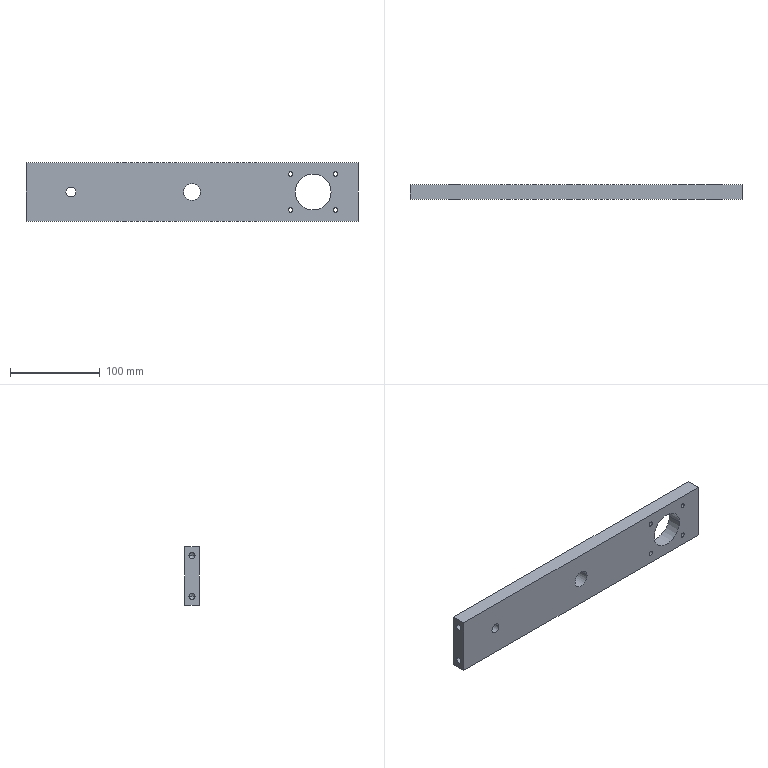Component | SolidWorks | BearingHousingMountingPlate-2 | 1 solid | 36 faces | box 370 x 16 x 65 mm | volume 354056 mm3 | cylinder 22 | cone 8 | plane 6 | commonest cylinder face diameters 5 x8 6.8 x8 19 x2 11 x2 40 x2
build123d program:
from build123d import *

# Parameters (mm, degrees)
SKETCH1_W             = 370
SKETCH1_H             = 65
SKETCH1_R             = 20
SKETCH1_R_2           = 5.5
SKETCH1_R_3           = 9.5
EXTRUDE1_DEPTH        = 16
M8_TAPPED_HOLE1_D     = 6.8
M8_TAPPED_HOLE1_DEPTH = 22.25
M8_TAPPED_HOLE1_TIP   = 2.043
M8_TAPPED_HOLE2_D     = 6.8
M8_TAPPED_HOLE2_DEPTH = 22.25
M8_TAPPED_HOLE2_TIP   = 2.043
M6_TAPPED_HOLE1_D     = 5
M6_TAPPED_HOLE1_DEPTH = 17
M6_TAPPED_HOLE1_TIP   = 1.502


with BuildPart() as part:
    # Sketch1 → Extrude1 (new body)
    with BuildSketch(Plane.XY):
        Rectangle(SKETCH1_W, SKETCH1_H)
        with Locations((135, 0)):
            Circle(SKETCH1_R, mode=Mode.SUBTRACT)
        with Locations((-135, 0)):
            Circle(SKETCH1_R_2, mode=Mode.SUBTRACT)
        Circle(SKETCH1_R_3, mode=Mode.SUBTRACT)
    extrude(amount=EXTRUDE1_DEPTH)

    # M8 Tapped Hole1
    with Locations(Plane(origin=(185, 22.5, 8), x_dir=(0, 0, 1), z_dir=(1, 0, 0))):
        with Locations((0, 0), (0, 45)):
            Hole(M8_TAPPED_HOLE1_D / 2, depth=M8_TAPPED_HOLE1_DEPTH)
            with Locations((0, 0, -(M8_TAPPED_HOLE1_DEPTH + M8_TAPPED_HOLE1_TIP / 2))):  # 118° drill point
                Cone(0, M8_TAPPED_HOLE1_D / 2, M8_TAPPED_HOLE1_TIP, mode=Mode.SUBTRACT)

    # M8 Tapped Hole2
    with Locations(Plane.ZY.offset(185)):
        with Locations((8, 22.5), (8, -22.5)):
            Hole(M8_TAPPED_HOLE2_D / 2, depth=M8_TAPPED_HOLE2_DEPTH)
            with Locations((0, 0, -(M8_TAPPED_HOLE2_DEPTH + M8_TAPPED_HOLE2_TIP / 2))):  # 118° drill point
                Cone(0, M8_TAPPED_HOLE2_D / 2, M8_TAPPED_HOLE2_TIP, mode=Mode.SUBTRACT)

    # M6 Tapped Hole1
    with Locations(Plane(origin=(0, 0, 0), x_dir=(-1, 0, 0), z_dir=(0, 0, -1))):
        with Locations((-110, -20), (-110, 20), (-160, 20), (-160, -20)):
            Hole(M6_TAPPED_HOLE1_D / 2, depth=M6_TAPPED_HOLE1_DEPTH)
            with Locations((0, 0, -(M6_TAPPED_HOLE1_DEPTH + M6_TAPPED_HOLE1_TIP / 2))):  # 118° drill point
                Cone(0, M6_TAPPED_HOLE1_D / 2, M6_TAPPED_HOLE1_TIP, mode=Mode.SUBTRACT)


solid = part.part

# Placed as in the assembly
solid = solid.moved(Location((250.217, 503.983, -28.052), (90, 0, 0)))